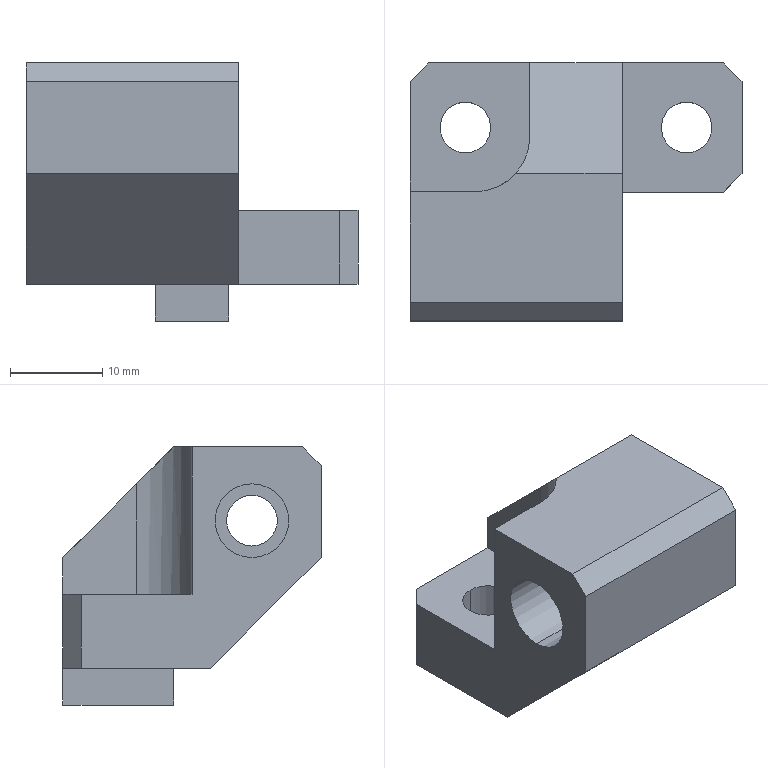Component | SolidWorks | 015GuideRodHolder-1 | 1 solid | 32 faces | box 36 x 28 x 28 mm | volume 10606 mm3 | plane 23 | cylinder 9 | commonest cylinder face diameters 5.5 x6 8 x2 12 x1
build123d program:
from build123d import *

# Parameters (mm, degrees)
SKETCH1_W                = 14
SKETCH1_H                = 36
EXTRUDE1_DEPTH           = 8
SKETCH3_W                = 28
SKETCH3_H                = 10
EXTRUDE3_DEPTH           = 16
M5_CLEARANCE_HOLE2_D     = 5.5
M5_CLEARANCE_HOLE2_DEPTH = 40
SKETCH7_R                = 4
CUT_EXTRUDE1_DEPTH       = 6
M5_CLEARANCE_HOLE1_D     = 5.5
M5_CLEARANCE_HOLE1_DEPTH = 23
SKETCH10_W               = 14
SKETCH10_H               = 10
EXTRUDE4_DEPTH           = 8
BOSS_EXTRUDE1_START      = 13
SKETCH12_W               = 14
SKETCH12_H               = 24
SKETCH12_R               = 4
BOSS_EXTRUDE1_DEPTH      = 13
FILLET1_R                = 6
SKETCH13_W               = 12
SKETCH13_H               = 8
BOSS_EXTRUDE2_DEPTH      = 4
FILLET1_OF_MIRROR3_R     = 6
SKETCH14_W               = 28
SKETCH14_H               = 28
CUT_EXTRUDE2_DEPTH       = 53.545
CHAMFER2_SIZE            = 2
CHAMFER3_SIZE            = 12
CHAMFER4_SIZE            = 2


with BuildPart() as part:
    # Sketch1 → Extrude1 (new body)
    with BuildSketch(Plane.XY):
        Rectangle(SKETCH1_W, SKETCH1_H)
    extrude1 = extrude(amount=EXTRUDE1_DEPTH)

    # Sketch3 → Extrude3 (add)
    with BuildSketch(Plane.XY.offset(8)):
        with Locations((7, 0)):
            Rectangle(SKETCH3_W, SKETCH3_H)
    extrude3 = extrude(amount=EXTRUDE3_DEPTH)

    # M5 Clearance Hole2
    with Locations(Plane.XY.offset(8)):
        with Locations((0, 12), (0, -12)):
            m5_clearance_hole2 = Hole(M5_CLEARANCE_HOLE2_D / 2, depth=M5_CLEARANCE_HOLE2_DEPTH)

    # Sketch7 → Cut-Extrude1 (cut)
    with BuildSketch(Plane(origin=(0, 5, 0), x_dir=(-1, 0, 0), z_dir=(0, 1, 0))):
        with Locations(Location((-13.5, 16, 0), (0, 0, 90))):
            Circle(SKETCH7_R)
    cut_extrude1 = extrude(amount=-CUT_EXTRUDE1_DEPTH, mode=Mode.SUBTRACT)

    # M5 Clearance Hole1
    with Locations(Plane(origin=(13.5, -5, 16), x_dir=(0, 0, -1), z_dir=(0, -1, 0))):
        with Locations((0, 0)):
            m5_clearance_hole1 = Hole(M5_CLEARANCE_HOLE1_D / 2, depth=M5_CLEARANCE_HOLE1_DEPTH)

    # Sketch10 → Extrude4 (add)
    with BuildSketch(Plane(origin=(0, 0, 8), x_dir=(-1, 0, 0), z_dir=(0, 0, -1))):
        with Locations((-14, 0)):
            Rectangle(SKETCH10_W, SKETCH10_H)
    extrude4 = extrude(amount=EXTRUDE4_DEPTH)

    # Sketch12 → Boss-Extrude1 (add)
    with BuildSketch(Plane(origin=(0, 5, 0), x_dir=(1, 0, 0), z_dir=(0, 1, 0)).offset(BOSS_EXTRUDE1_START)):
        with Locations((14, -12)):
            Rectangle(SKETCH12_W, SKETCH12_H)
        with Locations(Location((13.5, -16, 0), (0, 0, 270))):
            Circle(SKETCH12_R, mode=Mode.SUBTRACT)
    boss_extrude1 = extrude(amount=-BOSS_EXTRUDE1_DEPTH)

    # Fillet1
    fillet1_edges = [part.edges().sort_by_distance(p)[0] for p in [
        (7, 5, 16),
    ]]
    fillet(fillet1_edges, radius=FILLET1_R)

    # Sketch13 → Boss-Extrude2 (add)
    with BuildSketch(Plane(origin=(0, 0, 0), x_dir=(-1, 0, 0), z_dir=(0, 0, -1))):
        with Locations((1, 0)):
            Rectangle(SKETCH13_W, SKETCH13_H)
    boss_extrude2 = extrude(amount=BOSS_EXTRUDE2_DEPTH)

    # Mirror3: Extrude1, Extrude3, M5 Clearance Hole2, Cut-Extrude1, M5 Clearance Hole1, Extrude4, Boss-Extrude1, Boss-Extrude2 across plane
    add(extrude1.mirror(Plane.XY.offset(-4)))
    add(extrude3.mirror(Plane.XY.offset(-4)))
    add(m5_clearance_hole2.mirror(Plane.XY.offset(-4)), mode=Mode.SUBTRACT)
    add(cut_extrude1.mirror(Plane.XY.offset(-4)), mode=Mode.SUBTRACT)
    add(m5_clearance_hole1.mirror(Plane.XY.offset(-4)), mode=Mode.SUBTRACT)
    add(extrude4.mirror(Plane.XY.offset(-4)))
    add(boss_extrude1.mirror(Plane.XY.offset(-4)))
    add(boss_extrude2.mirror(Plane.XY.offset(-4)))

    # Fillet1 of Mirror3
    fillet1_of_mirror3_edges = [part.edges().sort_by_distance(p)[0] for p in [
        (7, 5, -24),
    ]]
    fillet(fillet1_of_mirror3_edges, radius=FILLET1_OF_MIRROR3_R)

    # Sketch14 → Cut-Extrude2 (cut, through all)
    with BuildSketch(Plane.XZ.offset(18)):
        with Locations((7, 10)):
            Rectangle(SKETCH14_W, SKETCH14_H)
    extrude(amount=-CUT_EXTRUDE2_DEPTH, mode=Mode.SUBTRACT)

    # Chamfer2
    chamfer2_edges = [part.edges().sort_by_distance(p)[0] for p in [
        (-7, 18, -12),
        (7, -18, -12),
        (-7, -18, -12),
    ]]
    chamfer(chamfer2_edges, length=CHAMFER2_SIZE)

    # Chamfer3
    chamfer3_edges = [part.edges().sort_by_distance(p)[0] for p in [
        (21, 6.5, -8),
        (-7, 0, -32),
    ]]
    chamfer(chamfer3_edges, length=CHAMFER3_SIZE)

    # Chamfer4
    chamfer4_edges = [part.edges().sort_by_distance(p)[0] for p in [
        (21, 6.5, -32),
    ]]
    chamfer(chamfer4_edges, length=CHAMFER4_SIZE)


solid = part.part

# Placed as in the assembly
solid = solid.moved(Location((25.76, 38.424, 29.04), (180, 0, 90)))
STEP:
#1=COLOUR_RGB('',0.7922,0.8196,0.9333);
#2=FILL_AREA_STYLE_COLOUR('',#1);
#3=FILL_AREA_STYLE('',(#2));
#4=SURFACE_STYLE_FILL_AREA(#3);
#5=SURFACE_SIDE_STYLE('',(#4));
#6=SURFACE_STYLE_USAGE(.BOTH.,#5);
#7=PRESENTATION_STYLE_ASSIGNMENT((#6));
#8=CARTESIAN_POINT('',(1.054,0.9813,2.196));
#9=VERTEX_POINT('',#8);
#10=CARTESIAN_POINT('',(1.054,0.9813,1.98));
#11=VERTEX_POINT('',#10);
#12=CARTESIAN_POINT('',(1.054,0.9813,2.088));
#13=DIRECTION('',(1.,0.,0.));
#14=DIRECTION('',(0.,0.,1.));
#15=AXIS2_PLACEMENT_3D('',#12,#13,#14);
#16=CIRCLE('',#15,0.1083);
#17=EDGE_CURVE('',#9,#11,#16,.T.);
#18=ORIENTED_EDGE('',*,*,#17,.F.);
#19=CARTESIAN_POINT('',(1.211,0.9813,2.196));
#20=VERTEX_POINT('',#19);
#21=CARTESIAN_POINT('',(1.211,0.9813,2.196));
#22=DIRECTION('',(1.,0.,0.));
#23=VECTOR('',#22,39.37);
#24=LINE('',#21,#23);
#25=EDGE_CURVE('',#9,#20,#24,.T.);
#26=ORIENTED_EDGE('',*,*,#25,.T.);
#27=CARTESIAN_POINT('',(1.211,0.9813,1.98));
#28=VERTEX_POINT('',#27);
#29=CARTESIAN_POINT('',(1.211,0.9813,2.088));
#30=DIRECTION('',(-1.,-0.,0.));
#31=DIRECTION('',(0.,0.,-1.));
#32=AXIS2_PLACEMENT_3D('',#29,#30,#31);
#33=CIRCLE('',#32,0.1083);
#34=EDGE_CURVE('',#28,#20,#33,.T.);
#35=ORIENTED_EDGE('',*,*,#34,.F.);
#36=CARTESIAN_POINT('',(1.211,0.9813,1.98));
#37=DIRECTION('',(1.,0.,0.));
#38=VECTOR('',#37,39.37);
#39=LINE('',#36,#38);
#40=EDGE_CURVE('',#11,#28,#39,.T.);
#41=ORIENTED_EDGE('',*,*,#40,.F.);
#42=EDGE_LOOP('',(#18,#26,#35,#41));
#43=FACE_OUTER_BOUND('',#42,.T.);
#44=CARTESIAN_POINT('',(1.211,0.9813,2.088));
#45=DIRECTION('',(1.,0.,0.));
#46=DIRECTION('',(0.,0.,-1.));
#47=AXIS2_PLACEMENT_3D('',#44,#45,#46);
#48=CYLINDRICAL_SURFACE('',#47,0.1083);
#49=ADVANCED_FACE('',(#43),#48,.F.);
#50=CARTESIAN_POINT('',(1.054,0.9813,2.246));
#51=VERTEX_POINT('',#50);
#52=CARTESIAN_POINT('',(1.054,0.9813,1.931));
#53=VERTEX_POINT('',#52);
#54=CARTESIAN_POINT('',(1.054,0.9813,2.088));
#55=DIRECTION('',(1.,0.,0.));
#56=DIRECTION('',(0.,0.,1.));
#57=AXIS2_PLACEMENT_3D('',#54,#55,#56);
#58=CIRCLE('',#57,0.1575);
#59=EDGE_CURVE('',#51,#53,#58,.T.);
#60=ORIENTED_EDGE('',*,*,#59,.T.);
#61=CARTESIAN_POINT('',(0.3055,0.9813,1.931));
#62=VERTEX_POINT('',#61);
#63=CARTESIAN_POINT('',(1.054,0.9813,1.931));
#64=DIRECTION('',(-1.,-0.,0.));
#65=VECTOR('',#64,39.37);
#66=LINE('',#63,#65);
#67=EDGE_CURVE('',#53,#62,#66,.T.);
#68=ORIENTED_EDGE('',*,*,#67,.T.);
#69=CARTESIAN_POINT('',(0.3055,0.9813,2.246));
#70=VERTEX_POINT('',#69);
#71=CARTESIAN_POINT('',(0.3055,0.9813,2.088));
#72=DIRECTION('',(-1.,-0.,0.));
#73=DIRECTION('',(-0.,0.,-1.));
#74=AXIS2_PLACEMENT_3D('',#71,#72,#73);
#75=CIRCLE('',#74,0.1575);
#76=EDGE_CURVE('',#62,#70,#75,.T.);
#77=ORIENTED_EDGE('',*,*,#76,.T.);
#78=CARTESIAN_POINT('',(1.054,0.9813,2.246));
#79=DIRECTION('',(-1.,-0.,0.));
#80=VECTOR('',#79,39.37);
#81=LINE('',#78,#80);
#82=EDGE_CURVE('',#51,#70,#81,.T.);
#83=ORIENTED_EDGE('',*,*,#82,.F.);
#84=EDGE_LOOP('',(#60,#68,#77,#83));
#85=FACE_OUTER_BOUND('',#84,.T.);
#86=CARTESIAN_POINT('',(1.054,0.9813,2.088));
#87=DIRECTION('',(-1.,-0.,0.));
#88=DIRECTION('',(0.,0.,1.));
#89=AXIS2_PLACEMENT_3D('',#86,#87,#88);
#90=CYLINDRICAL_SURFACE('',#89,0.1575);
#91=ADVANCED_FACE('',(#85),#90,.F.);
#92=CARTESIAN_POINT('',(0.5417,1.405,1.458));
#93=VERTEX_POINT('',#92);
#94=CARTESIAN_POINT('',(0.5417,1.621,1.458));
#95=VERTEX_POINT('',#94);
#96=CARTESIAN_POINT('',(0.5417,1.513,1.458));
#97=DIRECTION('',(-0.,0.,-1.));
#98=DIRECTION('',(0.,-1.,0.));
#99=AXIS2_PLACEMENT_3D('',#96,#97,#98);
#100=CIRCLE('',#99,0.1083);
#101=EDGE_CURVE('',#93,#95,#100,.T.);
#102=ORIENTED_EDGE('',*,*,#101,.T.);
#103=CARTESIAN_POINT('',(0.5417,1.621,1.773));
#104=VERTEX_POINT('',#103);
#105=CARTESIAN_POINT('',(0.5417,1.621,1.773));
#106=DIRECTION('',(0.,-0.,1.));
#107=VECTOR('',#106,39.37);
#108=LINE('',#105,#107);
#109=EDGE_CURVE('',#95,#104,#108,.T.);
#110=ORIENTED_EDGE('',*,*,#109,.T.);
#111=CARTESIAN_POINT('',(0.5417,1.405,1.773));
#112=VERTEX_POINT('',#111);
#113=CARTESIAN_POINT('',(0.5417,1.513,1.773));
#114=DIRECTION('',(-0.,0.,-1.));
#115=DIRECTION('',(0.,-1.,0.));
#116=AXIS2_PLACEMENT_3D('',#113,#114,#115);
#117=CIRCLE('',#116,0.1083);
#118=EDGE_CURVE('',#112,#104,#117,.T.);
#119=ORIENTED_EDGE('',*,*,#118,.F.);
#120=CARTESIAN_POINT('',(0.5417,1.405,1.773));
#121=DIRECTION('',(0.,-0.,1.));
#122=VECTOR('',#121,39.37);
#123=LINE('',#120,#122);
#124=EDGE_CURVE('',#93,#112,#123,.T.);
#125=ORIENTED_EDGE('',*,*,#124,.F.);
#126=EDGE_LOOP('',(#102,#110,#119,#125));
#127=FACE_OUTER_BOUND('',#126,.T.);
#128=CARTESIAN_POINT('',(0.5417,1.513,1.773));
#129=DIRECTION('',(0.,-0.,1.));
#130=DIRECTION('',(0.,-1.,0.));
#131=AXIS2_PLACEMENT_3D('',#128,#129,#130);
#132=CYLINDRICAL_SURFACE('',#131,0.1083);
#133=ADVANCED_FACE('',(#127),#132,.F.);
#134=CARTESIAN_POINT('',(1.487,1.405,1.458));
#135=VERTEX_POINT('',#134);
#136=CARTESIAN_POINT('',(1.487,1.621,1.458));
#137=VERTEX_POINT('',#136);
#138=CARTESIAN_POINT('',(1.487,1.513,1.458));
#139=DIRECTION('',(-0.,0.,-1.));
#140=DIRECTION('',(0.,-1.,0.));
#141=AXIS2_PLACEMENT_3D('',#138,#139,#140);
#142=CIRCLE('',#141,0.1083);
#143=EDGE_CURVE('',#135,#137,#142,.T.);
#144=ORIENTED_EDGE('',*,*,#143,.T.);
#145=CARTESIAN_POINT('',(1.487,1.621,1.773));
#146=VERTEX_POINT('',#145);
#147=CARTESIAN_POINT('',(1.487,1.621,1.773));
#148=DIRECTION('',(0.,-0.,1.));
#149=VECTOR('',#148,39.37);
#150=LINE('',#147,#149);
#151=EDGE_CURVE('',#137,#146,#150,.T.);
#152=ORIENTED_EDGE('',*,*,#151,.T.);
#153=CARTESIAN_POINT('',(1.487,1.405,1.773));
#154=VERTEX_POINT('',#153);
#155=CARTESIAN_POINT('',(1.487,1.513,1.773));
#156=DIRECTION('',(-0.,0.,-1.));
#157=DIRECTION('',(0.,-1.,0.));
#158=AXIS2_PLACEMENT_3D('',#155,#156,#157);
#159=CIRCLE('',#158,0.1083);
#160=EDGE_CURVE('',#154,#146,#159,.T.);
#161=ORIENTED_EDGE('',*,*,#160,.F.);
#162=CARTESIAN_POINT('',(1.487,1.405,1.773));
#163=DIRECTION('',(0.,-0.,1.));
#164=VECTOR('',#163,39.37);
#165=LINE('',#162,#164);
#166=EDGE_CURVE('',#135,#154,#165,.T.);
#167=ORIENTED_EDGE('',*,*,#166,.F.);
#168=EDGE_LOOP('',(#144,#152,#161,#167));
#169=FACE_OUTER_BOUND('',#168,.T.);
#170=CARTESIAN_POINT('',(1.487,1.513,1.773));
#171=DIRECTION('',(0.,-0.,1.));
#172=DIRECTION('',(0.,-1.,0.));
#173=AXIS2_PLACEMENT_3D('',#170,#171,#172);
#174=CYLINDRICAL_SURFACE('',#173,0.1083);
#175=ADVANCED_FACE('',(#169),#174,.F.);
#176=CARTESIAN_POINT('',(0.8173,1.788,1.931));
#177=VERTEX_POINT('',#176);
#178=CARTESIAN_POINT('',(0.8173,1.788,1.773));
#179=VERTEX_POINT('',#178);
#180=CARTESIAN_POINT('',(0.8173,1.788,2.403));
#181=DIRECTION('',(-0.,0.,-1.));
#182=VECTOR('',#181,39.37);
#183=LINE('',#180,#182);
#184=EDGE_CURVE('',#177,#179,#183,.T.);
#185=ORIENTED_EDGE('',*,*,#184,.F.);
#186=CARTESIAN_POINT('',(1.211,1.788,1.931));
#187=VERTEX_POINT('',#186);
#188=CARTESIAN_POINT('',(1.211,1.788,1.931));
#189=DIRECTION('',(1.,-0.,-0.));
#190=VECTOR('',#189,39.37);
#191=LINE('',#188,#190);
#192=EDGE_CURVE('',#177,#187,#191,.T.);
#193=ORIENTED_EDGE('',*,*,#192,.T.);
#194=CARTESIAN_POINT('',(1.211,1.788,1.773));
#195=VERTEX_POINT('',#194);
#196=CARTESIAN_POINT('',(1.211,1.788,2.403));
#197=DIRECTION('',(-0.,0.,-1.));
#198=VECTOR('',#197,39.37);
#199=LINE('',#196,#198);
#200=EDGE_CURVE('',#187,#195,#199,.T.);
#201=ORIENTED_EDGE('',*,*,#200,.T.);
#202=CARTESIAN_POINT('',(1.644,1.788,1.773));
#203=VERTEX_POINT('',#202);
#204=CARTESIAN_POINT('',(0.3055,1.788,1.773));
#205=DIRECTION('',(1.,-0.,-0.));
#206=VECTOR('',#205,39.37);
#207=LINE('',#204,#206);
#208=EDGE_CURVE('',#195,#203,#207,.T.);
#209=ORIENTED_EDGE('',*,*,#208,.T.);
#210=CARTESIAN_POINT('',(1.644,1.788,1.458));
#211=VERTEX_POINT('',#210);
#212=CARTESIAN_POINT('',(1.644,1.788,0.8284));
#213=DIRECTION('',(-0.,0.,-1.));
#214=VECTOR('',#213,39.37);
#215=LINE('',#212,#214);
#216=EDGE_CURVE('',#203,#211,#215,.T.);
#217=ORIENTED_EDGE('',*,*,#216,.T.);
#218=CARTESIAN_POINT('',(1.172,1.788,1.458));
#219=VERTEX_POINT('',#218);
#220=CARTESIAN_POINT('',(0.3055,1.788,1.458));
#221=DIRECTION('',(1.,-0.,-0.));
#222=VECTOR('',#221,39.37);
#223=LINE('',#220,#222);
#224=EDGE_CURVE('',#219,#211,#223,.T.);
#225=ORIENTED_EDGE('',*,*,#224,.F.);
#226=CARTESIAN_POINT('',(1.172,1.788,1.301));
#227=VERTEX_POINT('',#226);
#228=CARTESIAN_POINT('',(1.172,1.788,1.301));
#229=DIRECTION('',(-0.,0.,-1.));
#230=VECTOR('',#229,39.37);
#231=LINE('',#228,#230);
#232=EDGE_CURVE('',#219,#227,#231,.T.);
#233=ORIENTED_EDGE('',*,*,#232,.T.);
#234=CARTESIAN_POINT('',(0.8567,1.788,1.301));
#235=VERTEX_POINT('',#234);
#236=CARTESIAN_POINT('',(0.3055,1.788,1.301));
#237=DIRECTION('',(1.,0.,0.));
#238=VECTOR('',#237,39.37);
#239=LINE('',#236,#238);
#240=EDGE_CURVE('',#235,#227,#239,.T.);
#241=ORIENTED_EDGE('',*,*,#240,.F.);
#242=CARTESIAN_POINT('',(0.8567,1.788,1.458));
#243=VERTEX_POINT('',#242);
#244=CARTESIAN_POINT('',(0.8567,1.788,1.301));
#245=DIRECTION('',(-0.,0.,-1.));
#246=VECTOR('',#245,39.37);
#247=LINE('',#244,#246);
#248=EDGE_CURVE('',#243,#235,#247,.T.);
#249=ORIENTED_EDGE('',*,*,#248,.F.);
#250=CARTESIAN_POINT('',(0.3842,1.788,1.458));
#251=VERTEX_POINT('',#250);
#252=CARTESIAN_POINT('',(0.3055,1.788,1.458));
#253=DIRECTION('',(1.,-0.,-0.));
#254=VECTOR('',#253,39.37);
#255=LINE('',#252,#254);
#256=EDGE_CURVE('',#251,#243,#255,.T.);
#257=ORIENTED_EDGE('',*,*,#256,.F.);
#258=CARTESIAN_POINT('',(0.3842,1.788,1.773));
#259=VERTEX_POINT('',#258);
#260=CARTESIAN_POINT('',(0.3842,1.788,0.8284));
#261=DIRECTION('',(0.,-0.,1.));
#262=VECTOR('',#261,39.37);
#263=LINE('',#260,#262);
#264=EDGE_CURVE('',#251,#259,#263,.T.);
#265=ORIENTED_EDGE('',*,*,#264,.T.);
#266=CARTESIAN_POINT('',(0.3055,1.788,1.773));
#267=DIRECTION('',(1.,-0.,-0.));
#268=VECTOR('',#267,39.37);
#269=LINE('',#266,#268);
#270=EDGE_CURVE('',#259,#179,#269,.T.);
#271=ORIENTED_EDGE('',*,*,#270,.T.);
#272=EDGE_LOOP('',(#185,#193,#201,#209,#217,#225,#233,#241,#249,#257,#265,#271));
#273=FACE_OUTER_BOUND('',#272,.T.);
#274=CARTESIAN_POINT('',(0.3055,1.788,0.8284));
#275=DIRECTION('',(-0.,-1.,-0.));
#276=DIRECTION('',(-1.,0.,0.));
#277=AXIS2_PLACEMENT_3D('',#274,#275,#276);
#278=PLANE('',#277);
#279=ADVANCED_FACE('',(#273),#278,.F.);
#280=ORIENTED_EDGE('',*,*,#248,.T.);
#281=CARTESIAN_POINT('',(0.8567,1.316,1.301));
#282=VERTEX_POINT('',#281);
#283=CARTESIAN_POINT('',(0.8567,1.788,1.301));
#284=DIRECTION('',(0.,-1.,-0.));
#285=VECTOR('',#284,39.37);
#286=LINE('',#283,#285);
#287=EDGE_CURVE('',#235,#282,#286,.T.);
#288=ORIENTED_EDGE('',*,*,#287,.T.);
#289=CARTESIAN_POINT('',(0.8567,1.316,1.458));
#290=VERTEX_POINT('',#289);
#291=CARTESIAN_POINT('',(0.8567,1.316,1.301));
#292=DIRECTION('',(-0.,0.,-1.));
#293=VECTOR('',#292,39.37);
#294=LINE('',#291,#293);
#295=EDGE_CURVE('',#290,#282,#294,.T.);
#296=ORIENTED_EDGE('',*,*,#295,.F.);
#297=CARTESIAN_POINT('',(0.8567,1.788,1.458));
#298=DIRECTION('',(0.,-1.,-0.));
#299=VECTOR('',#298,39.37);
#300=LINE('',#297,#299);
#301=EDGE_CURVE('',#243,#290,#300,.T.);
#302=ORIENTED_EDGE('',*,*,#301,.F.);
#303=EDGE_LOOP('',(#280,#288,#296,#302));
#304=FACE_OUTER_BOUND('',#303,.T.);
#305=CARTESIAN_POINT('',(0.8567,1.788,1.301));
#306=DIRECTION('',(1.,0.,0.));
#307=DIRECTION('',(0.,-1.,-0.));
#308=AXIS2_PLACEMENT_3D('',#305,#306,#307);
#309=PLANE('',#308);
#310=ADVANCED_FACE('',(#304),#309,.F.);
#311=ORIENTED_EDGE('',*,*,#295,.T.);
#312=CARTESIAN_POINT('',(1.172,1.316,1.301));
#313=VERTEX_POINT('',#312);
#314=CARTESIAN_POINT('',(0.8567,1.316,1.301));
#315=DIRECTION('',(1.,0.,0.));
#316=VECTOR('',#315,39.37);
#317=LINE('',#314,#316);
#318=EDGE_CURVE('',#282,#313,#317,.T.);
#319=ORIENTED_EDGE('',*,*,#318,.T.);
#320=CARTESIAN_POINT('',(1.172,1.316,1.458));
#321=VERTEX_POINT('',#320);
#322=CARTESIAN_POINT('',(1.172,1.316,1.301));
#323=DIRECTION('',(-0.,0.,-1.));
#324=VECTOR('',#323,39.37);
#325=LINE('',#322,#324);
#326=EDGE_CURVE('',#321,#313,#325,.T.);
#327=ORIENTED_EDGE('',*,*,#326,.F.);
#328=CARTESIAN_POINT('',(0.8567,1.316,1.458));
#329=DIRECTION('',(1.,0.,0.));
#330=VECTOR('',#329,39.37);
#331=LINE('',#328,#330);
#332=EDGE_CURVE('',#290,#321,#331,.T.);
#333=ORIENTED_EDGE('',*,*,#332,.F.);
#334=EDGE_LOOP('',(#311,#319,#327,#333));
#335=FACE_OUTER_BOUND('',#334,.T.);
#336=CARTESIAN_POINT('',(0.8567,1.316,1.301));
#337=DIRECTION('',(-0.,1.,0.));
#338=DIRECTION('',(1.,0.,0.));
#339=AXIS2_PLACEMENT_3D('',#336,#337,#338);
#340=PLANE('',#339);
#341=ADVANCED_FACE('',(#335),#340,.F.);
#342=ORIENTED_EDGE('',*,*,#326,.T.);
#343=CARTESIAN_POINT('',(1.172,1.788,1.301));
#344=DIRECTION('',(-0.,1.,0.));
#345=VECTOR('',#344,39.37);
#346=LINE('',#343,#345);
#347=EDGE_CURVE('',#313,#227,#346,.T.);
#348=ORIENTED_EDGE('',*,*,#347,.T.);
#349=ORIENTED_EDGE('',*,*,#232,.F.);
#350=CARTESIAN_POINT('',(1.172,1.788,1.458));
#351=DIRECTION('',(-0.,1.,0.));
#352=VECTOR('',#351,39.37);
#353=LINE('',#350,#352);
#354=EDGE_CURVE('',#321,#219,#353,.T.);
#355=ORIENTED_EDGE('',*,*,#354,.F.);
#356=EDGE_LOOP('',(#342,#348,#349,#355));
#357=FACE_OUTER_BOUND('',#356,.T.);
#358=CARTESIAN_POINT('',(1.172,1.788,1.301));
#359=DIRECTION('',(-1.,-0.,-0.));
#360=DIRECTION('',(-0.,1.,0.));
#361=AXIS2_PLACEMENT_3D('',#358,#359,#360);
#362=PLANE('',#361);
#363=ADVANCED_FACE('',(#357),#362,.F.);
#364=ORIENTED_EDGE('',*,*,#143,.F.);
#365=CARTESIAN_POINT('',(1.487,1.513,1.458));
#366=DIRECTION('',(-0.,0.,-1.));
#367=DIRECTION('',(0.,-1.,0.));
#368=AXIS2_PLACEMENT_3D('',#365,#366,#367);
#369=CIRCLE('',#368,0.1083);
#370=EDGE_CURVE('',#137,#135,#369,.T.);
#371=ORIENTED_EDGE('',*,*,#370,.F.);
#372=EDGE_LOOP('',(#364,#371));
#373=FACE_BOUND('',#372,.T.);
#374=ORIENTED_EDGE('',*,*,#101,.F.);
#375=CARTESIAN_POINT('',(0.5417,1.513,1.458));
#376=DIRECTION('',(-0.,0.,-1.));
#377=DIRECTION('',(0.,-1.,0.));
#378=AXIS2_PLACEMENT_3D('',#375,#376,#377);
#379=CIRCLE('',#378,0.1083);
#380=EDGE_CURVE('',#95,#93,#379,.T.);
#381=ORIENTED_EDGE('',*,*,#380,.F.);
#382=EDGE_LOOP('',(#374,#381));
#383=FACE_BOUND('',#382,.T.);
#384=CARTESIAN_POINT('',(1.211,1.158,1.458));
#385=VERTEX_POINT('',#384);
#386=CARTESIAN_POINT('',(1.211,1.237,1.458));
#387=VERTEX_POINT('',#386);
#388=CARTESIAN_POINT('',(1.211,0.686,1.458));
#389=DIRECTION('',(-0.,1.,0.));
#390=VECTOR('',#389,39.37);
#391=LINE('',#388,#390);
#392=EDGE_CURVE('',#385,#387,#391,.T.);
#393=ORIENTED_EDGE('',*,*,#392,.F.);
#394=CARTESIAN_POINT('',(0.3055,1.158,1.458));
#395=VERTEX_POINT('',#394);
#396=CARTESIAN_POINT('',(1.723,1.158,1.458));
#397=DIRECTION('',(-1.,-0.,0.));
#398=VECTOR('',#397,39.37);
#399=LINE('',#396,#398);
#400=EDGE_CURVE('',#385,#395,#399,.T.);
#401=ORIENTED_EDGE('',*,*,#400,.T.);
#402=CARTESIAN_POINT('',(0.3055,1.71,1.458));
#403=VERTEX_POINT('',#402);
#404=CARTESIAN_POINT('',(0.3055,1.788,1.458));
#405=DIRECTION('',(-0.,1.,0.));
#406=VECTOR('',#405,39.37);
#407=LINE('',#404,#406);
#408=EDGE_CURVE('',#395,#403,#407,.T.);
#409=ORIENTED_EDGE('',*,*,#408,.T.);
#410=CARTESIAN_POINT('',(0.3055,1.71,1.458));
#411=DIRECTION('',(0.7071,0.7071,0.));
#412=VECTOR('',#411,39.37);
#413=LINE('',#410,#412);
#414=EDGE_CURVE('',#403,#251,#413,.T.);
#415=ORIENTED_EDGE('',*,*,#414,.T.);
#416=ORIENTED_EDGE('',*,*,#256,.T.);
#417=ORIENTED_EDGE('',*,*,#301,.T.);
#418=ORIENTED_EDGE('',*,*,#332,.T.);
#419=ORIENTED_EDGE('',*,*,#354,.T.);
#420=ORIENTED_EDGE('',*,*,#224,.T.);
#421=CARTESIAN_POINT('',(1.723,1.71,1.458));
#422=VERTEX_POINT('',#421);
#423=CARTESIAN_POINT('',(1.644,1.788,1.458));
#424=DIRECTION('',(0.7071,-0.7071,-0.));
#425=VECTOR('',#424,39.37);
#426=LINE('',#423,#425);
#427=EDGE_CURVE('',#211,#422,#426,.T.);
#428=ORIENTED_EDGE('',*,*,#427,.T.);
#429=CARTESIAN_POINT('',(1.723,1.316,1.458));
#430=VERTEX_POINT('',#429);
#431=CARTESIAN_POINT('',(1.723,1.788,1.458));
#432=DIRECTION('',(0.,-1.,-0.));
#433=VECTOR('',#432,39.37);
#434=LINE('',#431,#433);
#435=EDGE_CURVE('',#422,#430,#434,.T.);
#436=ORIENTED_EDGE('',*,*,#435,.T.);
#437=CARTESIAN_POINT('',(1.644,1.237,1.458));
#438=VERTEX_POINT('',#437);
#439=CARTESIAN_POINT('',(1.723,1.316,1.458));
#440=DIRECTION('',(-0.7071,-0.7071,-0.));
#441=VECTOR('',#440,39.37);
#442=LINE('',#439,#441);
#443=EDGE_CURVE('',#430,#438,#442,.T.);
#444=ORIENTED_EDGE('',*,*,#443,.T.);
#445=CARTESIAN_POINT('',(0.3055,1.237,1.458));
#446=DIRECTION('',(-1.,0.,0.));
#447=VECTOR('',#446,39.37);
#448=LINE('',#445,#447);
#449=EDGE_CURVE('',#438,#387,#448,.T.);
#450=ORIENTED_EDGE('',*,*,#449,.T.);
#451=EDGE_LOOP('',(#393,#401,#409,#415,#416,#417,#418,#419,#420,#428,#436,#444,#450));
#452=FACE_OUTER_BOUND('',#451,.T.);
#453=CARTESIAN_POINT('',(1.723,1.788,1.458));
#454=DIRECTION('',(0.,-0.,1.));
#455=DIRECTION('',(0.,-1.,-0.));
#456=AXIS2_PLACEMENT_3D('',#453,#454,#455);
#457=PLANE('',#456);
#458=ADVANCED_FACE('',(#373,#383,#452),#457,.F.);
#459=CARTESIAN_POINT('',(0.8173,1.473,2.246));
#460=VERTEX_POINT('',#459);
#461=CARTESIAN_POINT('',(0.8173,1.473,1.773));
#462=VERTEX_POINT('',#461);
#463=CARTESIAN_POINT('',(0.8173,1.473,1.773));
#464=DIRECTION('',(-0.,0.,-1.));
#465=VECTOR('',#464,39.37);
#466=LINE('',#463,#465);
#467=EDGE_CURVE('',#460,#462,#466,.T.);
#468=ORIENTED_EDGE('',*,*,#467,.F.);
#469=CARTESIAN_POINT('',(0.8173,1.788,1.931));
#470=DIRECTION('',(-0.,0.7071,-0.7071));
#471=VECTOR('',#470,39.37);
#472=LINE('',#469,#471);
#473=EDGE_CURVE('',#460,#177,#472,.T.);
#474=ORIENTED_EDGE('',*,*,#473,.T.);
#475=ORIENTED_EDGE('',*,*,#184,.T.);
#476=CARTESIAN_POINT('',(0.8173,1.788,1.773));
#477=DIRECTION('',(-0.,1.,0.));
#478=VECTOR('',#477,39.37);
#479=LINE('',#476,#478);
#480=EDGE_CURVE('',#462,#179,#479,.T.);
#481=ORIENTED_EDGE('',*,*,#480,.F.);
#482=EDGE_LOOP('',(#468,#474,#475,#481));
#483=FACE_OUTER_BOUND('',#482,.T.);
#484=CARTESIAN_POINT('',(0.8173,1.788,2.403));
#485=DIRECTION('',(1.,0.,-0.));
#486=DIRECTION('',(-0.,0.,-1.));
#487=AXIS2_PLACEMENT_3D('',#484,#485,#486);
#488=PLANE('',#487);
#489=ADVANCED_FACE('',(#483),#488,.F.);
#490=ORIENTED_EDGE('',*,*,#449,.F.);
#491=CARTESIAN_POINT('',(1.644,1.237,1.773));
#492=VERTEX_POINT('',#491);
#493=CARTESIAN_POINT('',(1.644,1.237,1.773));
#494=DIRECTION('',(0.,-0.,1.));
#495=VECTOR('',#494,39.37);
#496=LINE('',#493,#495);
#497=EDGE_CURVE('',#438,#492,#496,.T.);
#498=ORIENTED_EDGE('',*,*,#497,.T.);
#499=CARTESIAN_POINT('',(1.211,1.237,1.773));
#500=VERTEX_POINT('',#499);
#501=CARTESIAN_POINT('',(0.3055,1.237,1.773));
#502=DIRECTION('',(-1.,0.,0.));
#503=VECTOR('',#502,39.37);
#504=LINE('',#501,#503);
#505=EDGE_CURVE('',#492,#500,#504,.T.);
#506=ORIENTED_EDGE('',*,*,#505,.T.);
#507=CARTESIAN_POINT('',(1.211,1.237,1.458));
#508=DIRECTION('',(0.,-0.,1.));
#509=VECTOR('',#508,39.37);
#510=LINE('',#507,#509);
#511=EDGE_CURVE('',#387,#500,#510,.T.);
#512=ORIENTED_EDGE('',*,*,#511,.F.);
#513=EDGE_LOOP('',(#490,#498,#506,#512));
#514=FACE_OUTER_BOUND('',#513,.T.);
#515=CARTESIAN_POINT('',(0.3055,1.237,1.773));
#516=DIRECTION('',(0.,1.,0.));
#517=DIRECTION('',(1.,-0.,-0.));
#518=AXIS2_PLACEMENT_3D('',#515,#516,#517);
#519=PLANE('',#518);
#520=ADVANCED_FACE('',(#514),#519,.F.);
#521=ORIENTED_EDGE('',*,*,#118,.T.);
#522=CARTESIAN_POINT('',(0.5417,1.513,1.773));
#523=DIRECTION('',(-0.,0.,-1.));
#524=DIRECTION('',(0.,-1.,0.));
#525=AXIS2_PLACEMENT_3D('',#522,#523,#524);
#526=CIRCLE('',#525,0.1083);
#527=EDGE_CURVE('',#104,#112,#526,.T.);
#528=ORIENTED_EDGE('',*,*,#527,.T.);
#529=EDGE_LOOP('',(#521,#528));
#530=FACE_BOUND('',#529,.T.);
#531=ORIENTED_EDGE('',*,*,#270,.F.);
#532=CARTESIAN_POINT('',(0.3055,1.71,1.773));
#533=VERTEX_POINT('',#532);
#534=CARTESIAN_POINT('',(1.054,2.458,1.773));
#535=DIRECTION('',(-0.7071,-0.7071,-0.));
#536=VECTOR('',#535,39.37);
#537=LINE('',#534,#536);
#538=EDGE_CURVE('',#259,#533,#537,.T.);
#539=ORIENTED_EDGE('',*,*,#538,.T.);
#540=CARTESIAN_POINT('',(0.3055,1.237,1.773));
#541=VERTEX_POINT('',#540);
#542=CARTESIAN_POINT('',(0.3055,1.788,1.773));
#543=DIRECTION('',(-0.,1.,0.));
#544=VECTOR('',#543,39.37);
#545=LINE('',#542,#544);
#546=EDGE_CURVE('',#541,#533,#545,.T.);
#547=ORIENTED_EDGE('',*,*,#546,.F.);
#548=CARTESIAN_POINT('',(0.5811,1.237,1.773));
#549=VERTEX_POINT('',#548);
#550=CARTESIAN_POINT('',(0.3055,1.237,1.773));
#551=DIRECTION('',(-1.,0.,0.));
#552=VECTOR('',#551,39.37);
#553=LINE('',#550,#552);
#554=EDGE_CURVE('',#549,#541,#553,.T.);
#555=ORIENTED_EDGE('',*,*,#554,.F.);
#556=CARTESIAN_POINT('',(0.5811,1.473,1.773));
#557=DIRECTION('',(-0.,0.,-1.));
#558=DIRECTION('',(0.,-1.,0.));
#559=AXIS2_PLACEMENT_3D('',#556,#557,#558);
#560=CIRCLE('',#559,0.2362);
#561=EDGE_CURVE('',#462,#549,#560,.T.);
#562=ORIENTED_EDGE('',*,*,#561,.F.);
#563=ORIENTED_EDGE('',*,*,#480,.T.);
#564=EDGE_LOOP('',(#531,#539,#547,#555,#562,#563));
#565=FACE_OUTER_BOUND('',#564,.T.);
#566=CARTESIAN_POINT('',(1.723,1.788,1.773));
#567=DIRECTION('',(0.,-0.,1.));
#568=DIRECTION('',(0.,-1.,-0.));
#569=AXIS2_PLACEMENT_3D('',#566,#567,#568);
#570=PLANE('',#569);
#571=ADVANCED_FACE('',(#530,#565),#570,.T.);
#572=CARTESIAN_POINT('',(1.723,1.71,1.773));
#573=VERTEX_POINT('',#572);
#574=CARTESIAN_POINT('',(1.723,1.316,1.773));
#575=VERTEX_POINT('',#574);
#576=CARTESIAN_POINT('',(1.723,1.788,1.773));
#577=DIRECTION('',(0.,-1.,-0.));
#578=VECTOR('',#577,39.37);
#579=LINE('',#576,#578);
#580=EDGE_CURVE('',#573,#575,#579,.T.);
#581=ORIENTED_EDGE('',*,*,#580,.T.);
#582=CARTESIAN_POINT('',(1.723,1.316,1.773));
#583=DIRECTION('',(-0.,0.,-1.));
#584=VECTOR('',#583,39.37);
#585=LINE('',#582,#584);
#586=EDGE_CURVE('',#575,#430,#585,.T.);
#587=ORIENTED_EDGE('',*,*,#586,.T.);
#588=ORIENTED_EDGE('',*,*,#435,.F.);
#589=CARTESIAN_POINT('',(1.723,1.71,1.773));
#590=DIRECTION('',(0.,-0.,1.));
#591=VECTOR('',#590,39.37);
#592=LINE('',#589,#591);
#593=EDGE_CURVE('',#422,#573,#592,.T.);
#594=ORIENTED_EDGE('',*,*,#593,.T.);
#595=EDGE_LOOP('',(#581,#587,#588,#594));
#596=FACE_OUTER_BOUND('',#595,.T.);
#597=CARTESIAN_POINT('',(1.723,1.788,1.773));
#598=DIRECTION('',(-1.,-0.,0.));
#599=DIRECTION('',(0.,-0.,1.));
#600=AXIS2_PLACEMENT_3D('',#597,#598,#599);
#601=PLANE('',#600);
#602=ADVANCED_FACE('',(#596),#601,.F.);
#603=CARTESIAN_POINT('',(0.3055,0.686,1.931));
#604=VERTEX_POINT('',#603);
#605=CARTESIAN_POINT('',(0.3055,0.686,2.324));
#606=VERTEX_POINT('',#605);
#607=CARTESIAN_POINT('',(0.3055,0.686,1.458));
#608=DIRECTION('',(0.,-0.,1.));
#609=VECTOR('',#608,39.37);
#610=LINE('',#607,#609);
#611=EDGE_CURVE('',#604,#606,#610,.T.);
#612=ORIENTED_EDGE('',*,*,#611,.T.);
#613=CARTESIAN_POINT('',(0.3055,0.7647,2.403));
#614=VERTEX_POINT('',#613);
#615=CARTESIAN_POINT('',(0.3055,0.686,2.324));
#616=DIRECTION('',(0.,0.7071,0.7071));
#617=VECTOR('',#616,39.37);
#618=LINE('',#615,#617);
#619=EDGE_CURVE('',#606,#614,#618,.T.);
#620=ORIENTED_EDGE('',*,*,#619,.T.);
#621=CARTESIAN_POINT('',(0.3055,1.237,2.403));
#622=VERTEX_POINT('',#621);
#623=CARTESIAN_POINT('',(0.3055,0.686,2.403));
#624=DIRECTION('',(-0.,1.,0.));
#625=VECTOR('',#624,39.37);
#626=LINE('',#623,#625);
#627=EDGE_CURVE('',#614,#622,#626,.T.);
#628=ORIENTED_EDGE('',*,*,#627,.T.);
#629=CARTESIAN_POINT('',(0.3055,1.237,1.458));
#630=DIRECTION('',(-0.,0.,-1.));
#631=VECTOR('',#630,39.37);
#632=LINE('',#629,#631);
#633=EDGE_CURVE('',#622,#541,#632,.T.);
#634=ORIENTED_EDGE('',*,*,#633,.T.);
#635=ORIENTED_EDGE('',*,*,#546,.T.);
#636=CARTESIAN_POINT('',(0.3055,1.71,1.773));
#637=DIRECTION('',(-0.,0.,-1.));
#638=VECTOR('',#637,39.37);
#639=LINE('',#636,#638);
#640=EDGE_CURVE('',#533,#403,#639,.T.);
#641=ORIENTED_EDGE('',*,*,#640,.T.);
#642=ORIENTED_EDGE('',*,*,#408,.F.);
#643=CARTESIAN_POINT('',(0.3055,0.686,1.931));
#644=DIRECTION('',(0.,-0.7071,0.7071));
#645=VECTOR('',#644,39.37);
#646=LINE('',#643,#645);
#647=EDGE_CURVE('',#395,#604,#646,.T.);
#648=ORIENTED_EDGE('',*,*,#647,.T.);
#649=EDGE_LOOP('',(#612,#620,#628,#634,#635,#641,#642,#648));
#650=FACE_OUTER_BOUND('',#649,.T.);
#651=CARTESIAN_POINT('',(0.3055,0.9813,2.088));
#652=DIRECTION('',(-1.,-0.,0.));
#653=DIRECTION('',(-0.,0.,-1.));
#654=AXIS2_PLACEMENT_3D('',#651,#652,#653);
#655=CIRCLE('',#654,0.1575);
#656=EDGE_CURVE('',#70,#62,#655,.T.);
#657=ORIENTED_EDGE('',*,*,#656,.F.);
#658=ORIENTED_EDGE('',*,*,#76,.F.);
#659=EDGE_LOOP('',(#657,#658));
#660=FACE_BOUND('',#659,.T.);
#661=CARTESIAN_POINT('',(0.3055,1.788,1.773));
#662=DIRECTION('',(1.,0.,-0.));
#663=DIRECTION('',(-0.,0.,-1.));
#664=AXIS2_PLACEMENT_3D('',#661,#662,#663);
#665=PLANE('',#664);
#666=ADVANCED_FACE('',(#650,#660),#665,.F.);
#667=ORIENTED_EDGE('',*,*,#160,.T.);
#668=CARTESIAN_POINT('',(1.487,1.513,1.773));
#669=DIRECTION('',(-0.,0.,-1.));
#670=DIRECTION('',(0.,-1.,0.));
#671=AXIS2_PLACEMENT_3D('',#668,#669,#670);
#672=CIRCLE('',#671,0.1083);
#673=EDGE_CURVE('',#146,#154,#672,.T.);
#674=ORIENTED_EDGE('',*,*,#673,.T.);
#675=EDGE_LOOP('',(#667,#674));
#676=FACE_BOUND('',#675,.T.);
#677=ORIENTED_EDGE('',*,*,#505,.F.);
#678=CARTESIAN_POINT('',(1.959,1.552,1.773));
#679=DIRECTION('',(0.7071,0.7071,0.));
#680=VECTOR('',#679,39.37);
#681=LINE('',#678,#680);
#682=EDGE_CURVE('',#492,#575,#681,.T.);
#683=ORIENTED_EDGE('',*,*,#682,.T.);
#684=ORIENTED_EDGE('',*,*,#580,.F.);
#685=CARTESIAN_POINT('',(1.683,1.749,1.773));
#686=DIRECTION('',(-0.7071,0.7071,0.));
#687=VECTOR('',#686,39.37);
#688=LINE('',#685,#687);
#689=EDGE_CURVE('',#573,#203,#688,.T.);
#690=ORIENTED_EDGE('',*,*,#689,.T.);
#691=ORIENTED_EDGE('',*,*,#208,.F.);
#692=CARTESIAN_POINT('',(1.211,1.788,1.773));
#693=DIRECTION('',(0.,-1.,-0.));
#694=VECTOR('',#693,39.37);
#695=LINE('',#692,#694);
#696=EDGE_CURVE('',#195,#500,#695,.T.);
#697=ORIENTED_EDGE('',*,*,#696,.T.);
#698=EDGE_LOOP('',(#677,#683,#684,#690,#691,#697));
#699=FACE_OUTER_BOUND('',#698,.T.);
#700=CARTESIAN_POINT('',(1.723,1.788,1.773));
#701=DIRECTION('',(0.,-0.,1.));
#702=DIRECTION('',(0.,-1.,-0.));
#703=AXIS2_PLACEMENT_3D('',#700,#701,#702);
#704=PLANE('',#703);
#705=ADVANCED_FACE('',(#676,#699),#704,.T.);
#706=ORIENTED_EDGE('',*,*,#34,.T.);
#707=CARTESIAN_POINT('',(1.211,0.9813,2.088));
#708=DIRECTION('',(-1.,-0.,0.));
#709=DIRECTION('',(0.,0.,-1.));
#710=AXIS2_PLACEMENT_3D('',#707,#708,#709);
#711=CIRCLE('',#710,0.1083);
#712=EDGE_CURVE('',#20,#28,#711,.T.);
#713=ORIENTED_EDGE('',*,*,#712,.T.);
#714=EDGE_LOOP('',(#706,#713));
#715=FACE_BOUND('',#714,.T.);
#716=CARTESIAN_POINT('',(1.211,1.316,2.403));
#717=VERTEX_POINT('',#716);
#718=CARTESIAN_POINT('',(1.211,0.7647,2.403));
#719=VERTEX_POINT('',#718);
#720=CARTESIAN_POINT('',(1.211,1.788,2.403));
#721=DIRECTION('',(0.,-1.,-0.));
#722=VECTOR('',#721,39.37);
#723=LINE('',#720,#722);
#724=EDGE_CURVE('',#717,#719,#723,.T.);
#725=ORIENTED_EDGE('',*,*,#724,.T.);
#726=CARTESIAN_POINT('',(1.211,0.686,2.324));
#727=VERTEX_POINT('',#726);
#728=CARTESIAN_POINT('',(1.211,0.686,2.324));
#729=DIRECTION('',(-0.,-0.7071,-0.7071));
#730=VECTOR('',#729,39.37);
#731=LINE('',#728,#730);
#732=EDGE_CURVE('',#719,#727,#731,.T.);
#733=ORIENTED_EDGE('',*,*,#732,.T.);
#734=CARTESIAN_POINT('',(1.211,0.686,1.931));
#735=VERTEX_POINT('',#734);
#736=CARTESIAN_POINT('',(1.211,0.686,2.403));
#737=DIRECTION('',(-0.,0.,-1.));
#738=VECTOR('',#737,39.37);
#739=LINE('',#736,#738);
#740=EDGE_CURVE('',#727,#735,#739,.T.);
#741=ORIENTED_EDGE('',*,*,#740,.T.);
#742=CARTESIAN_POINT('',(1.211,0.686,1.931));
#743=DIRECTION('',(-0.,0.7071,-0.7071));
#744=VECTOR('',#743,39.37);
#745=LINE('',#742,#744);
#746=EDGE_CURVE('',#735,#385,#745,.T.);
#747=ORIENTED_EDGE('',*,*,#746,.T.);
#748=ORIENTED_EDGE('',*,*,#392,.T.);
#749=ORIENTED_EDGE('',*,*,#511,.T.);
#750=ORIENTED_EDGE('',*,*,#696,.F.);
#751=ORIENTED_EDGE('',*,*,#200,.F.);
#752=CARTESIAN_POINT('',(1.211,1.788,1.931));
#753=DIRECTION('',(0.,-0.7071,0.7071));
#754=VECTOR('',#753,39.37);
#755=LINE('',#752,#754);
#756=EDGE_CURVE('',#187,#717,#755,.T.);
#757=ORIENTED_EDGE('',*,*,#756,.T.);
#758=EDGE_LOOP('',(#725,#733,#741,#747,#748,#749,#750,#751,#757));
#759=FACE_OUTER_BOUND('',#758,.T.);
#760=CARTESIAN_POINT('',(1.211,1.788,2.403));
#761=DIRECTION('',(-1.,-0.,0.));
#762=DIRECTION('',(0.,-0.,1.));
#763=AXIS2_PLACEMENT_3D('',#760,#761,#762);
#764=PLANE('',#763);
#765=ADVANCED_FACE('',(#715,#759),#764,.F.);
#766=ORIENTED_EDGE('',*,*,#740,.F.);
#767=CARTESIAN_POINT('',(0.3055,0.686,2.324));
#768=DIRECTION('',(-1.,-0.,0.));
#769=VECTOR('',#768,39.37);
#770=LINE('',#767,#769);
#771=EDGE_CURVE('',#727,#606,#770,.T.);
#772=ORIENTED_EDGE('',*,*,#771,.T.);
#773=ORIENTED_EDGE('',*,*,#611,.F.);
#774=CARTESIAN_POINT('',(0.8173,0.686,1.931));
#775=DIRECTION('',(1.,0.,0.));
#776=VECTOR('',#775,39.37);
#777=LINE('',#774,#776);
#778=EDGE_CURVE('',#604,#735,#777,.T.);
#779=ORIENTED_EDGE('',*,*,#778,.T.);
#780=EDGE_LOOP('',(#766,#772,#773,#779));
#781=FACE_OUTER_BOUND('',#780,.T.);
#782=CARTESIAN_POINT('',(0.8173,0.686,2.403));
#783=DIRECTION('',(-0.,1.,0.));
#784=DIRECTION('',(0.,-0.,1.));
#785=AXIS2_PLACEMENT_3D('',#782,#783,#784);
#786=PLANE('',#785);
#787=ADVANCED_FACE('',(#781),#786,.F.);
#788=ORIENTED_EDGE('',*,*,#627,.F.);
#789=CARTESIAN_POINT('',(1.211,0.7647,2.403));
#790=DIRECTION('',(1.,0.,0.));
#791=VECTOR('',#790,39.37);
#792=LINE('',#789,#791);
#793=EDGE_CURVE('',#614,#719,#792,.T.);
#794=ORIENTED_EDGE('',*,*,#793,.T.);
#795=ORIENTED_EDGE('',*,*,#724,.F.);
#796=CARTESIAN_POINT('',(0.7572,1.316,2.403));
#797=VERTEX_POINT('',#796);
#798=CARTESIAN_POINT('',(0.8173,1.316,2.403));
#799=DIRECTION('',(-1.,0.,0.));
#800=VECTOR('',#799,39.37);
#801=LINE('',#798,#800);
#802=EDGE_CURVE('',#717,#797,#801,.T.);
#803=ORIENTED_EDGE('',*,*,#802,.T.);
#804=CARTESIAN_POINT('',(0.5811,1.237,2.403));
#805=VERTEX_POINT('',#804);
#806=CARTESIAN_POINT('',(0.5811,1.473,2.403));
#807=DIRECTION('',(0.,-0.,1.));
#808=DIRECTION('',(0.,-1.,0.));
#809=AXIS2_PLACEMENT_3D('',#806,#807,#808);
#810=CIRCLE('',#809,0.2362);
#811=EDGE_CURVE('',#805,#797,#810,.T.);
#812=ORIENTED_EDGE('',*,*,#811,.F.);
#813=CARTESIAN_POINT('',(-0.7884,1.237,2.403));
#814=DIRECTION('',(1.,0.,0.));
#815=VECTOR('',#814,39.37);
#816=LINE('',#813,#815);
#817=EDGE_CURVE('',#622,#805,#816,.T.);
#818=ORIENTED_EDGE('',*,*,#817,.F.);
#819=EDGE_LOOP('',(#788,#794,#795,#803,#812,#818));
#820=FACE_OUTER_BOUND('',#819,.T.);
#821=CARTESIAN_POINT('',(1.211,1.788,2.403));
#822=DIRECTION('',(0.,-0.,1.));
#823=DIRECTION('',(0.,-1.,-0.));
#824=AXIS2_PLACEMENT_3D('',#821,#822,#823);
#825=PLANE('',#824);
#826=ADVANCED_FACE('',(#820),#825,.T.);
#827=ORIENTED_EDGE('',*,*,#151,.F.);
#828=ORIENTED_EDGE('',*,*,#370,.T.);
#829=ORIENTED_EDGE('',*,*,#166,.T.);
#830=ORIENTED_EDGE('',*,*,#673,.F.);
#831=EDGE_LOOP('',(#827,#828,#829,#830));
#832=FACE_OUTER_BOUND('',#831,.T.);
#833=CARTESIAN_POINT('',(1.487,1.513,1.773));
#834=DIRECTION('',(0.,-0.,1.));
#835=DIRECTION('',(0.,-1.,0.));
#836=AXIS2_PLACEMENT_3D('',#833,#834,#835);
#837=CYLINDRICAL_SURFACE('',#836,0.1083);
#838=ADVANCED_FACE('',(#832),#837,.F.);
#839=ORIENTED_EDGE('',*,*,#109,.F.);
#840=ORIENTED_EDGE('',*,*,#380,.T.);
#841=ORIENTED_EDGE('',*,*,#124,.T.);
#842=ORIENTED_EDGE('',*,*,#527,.F.);
#843=EDGE_LOOP('',(#839,#840,#841,#842));
#844=FACE_OUTER_BOUND('',#843,.T.);
#845=CARTESIAN_POINT('',(0.5417,1.513,1.773));
#846=DIRECTION('',(0.,-0.,1.));
#847=DIRECTION('',(0.,-1.,0.));
#848=AXIS2_PLACEMENT_3D('',#845,#846,#847);
#849=CYLINDRICAL_SURFACE('',#848,0.1083);
#850=ADVANCED_FACE('',(#844),#849,.F.);
#851=ORIENTED_EDGE('',*,*,#67,.F.);
#852=CARTESIAN_POINT('',(1.054,0.9813,2.088));
#853=DIRECTION('',(1.,0.,0.));
#854=DIRECTION('',(0.,0.,1.));
#855=AXIS2_PLACEMENT_3D('',#852,#853,#854);
#856=CIRCLE('',#855,0.1575);
#857=EDGE_CURVE('',#53,#51,#856,.T.);
#858=ORIENTED_EDGE('',*,*,#857,.T.);
#859=ORIENTED_EDGE('',*,*,#82,.T.);
#860=ORIENTED_EDGE('',*,*,#656,.T.);
#861=EDGE_LOOP('',(#851,#858,#859,#860));
#862=FACE_OUTER_BOUND('',#861,.T.);
#863=CARTESIAN_POINT('',(1.054,0.9813,2.088));
#864=DIRECTION('',(-1.,-0.,0.));
#865=DIRECTION('',(0.,0.,1.));
#866=AXIS2_PLACEMENT_3D('',#863,#864,#865);
#867=CYLINDRICAL_SURFACE('',#866,0.1575);
#868=ADVANCED_FACE('',(#862),#867,.F.);
#869=CARTESIAN_POINT('',(1.054,0.9813,2.088));
#870=DIRECTION('',(1.,0.,0.));
#871=DIRECTION('',(0.,0.,1.));
#872=AXIS2_PLACEMENT_3D('',#869,#870,#871);
#873=CIRCLE('',#872,0.1083);
#874=EDGE_CURVE('',#11,#9,#873,.T.);
#875=ORIENTED_EDGE('',*,*,#874,.T.);
#876=ORIENTED_EDGE('',*,*,#17,.T.);
#877=EDGE_LOOP('',(#875,#876));
#878=FACE_BOUND('',#877,.T.);
#879=ORIENTED_EDGE('',*,*,#59,.F.);
#880=ORIENTED_EDGE('',*,*,#857,.F.);
#881=EDGE_LOOP('',(#879,#880));
#882=FACE_OUTER_BOUND('',#881,.T.);
#883=CARTESIAN_POINT('',(1.054,0.9813,2.088));
#884=DIRECTION('',(-1.,-0.,0.));
#885=DIRECTION('',(0.,-0.,1.));
#886=AXIS2_PLACEMENT_3D('',#883,#884,#885);
#887=PLANE('',#886);
#888=ADVANCED_FACE('',(#878,#882),#887,.T.);
#889=ORIENTED_EDGE('',*,*,#25,.F.);
#890=ORIENTED_EDGE('',*,*,#874,.F.);
#891=ORIENTED_EDGE('',*,*,#40,.T.);
#892=ORIENTED_EDGE('',*,*,#712,.F.);
#893=EDGE_LOOP('',(#889,#890,#891,#892));
#894=FACE_OUTER_BOUND('',#893,.T.);
#895=CARTESIAN_POINT('',(1.211,0.9813,2.088));
#896=DIRECTION('',(1.,0.,0.));
#897=DIRECTION('',(0.,0.,-1.));
#898=AXIS2_PLACEMENT_3D('',#895,#896,#897);
#899=CYLINDRICAL_SURFACE('',#898,0.1083);
#900=ADVANCED_FACE('',(#894),#899,.F.);
#901=ORIENTED_EDGE('',*,*,#554,.T.);
#902=ORIENTED_EDGE('',*,*,#633,.F.);
#903=ORIENTED_EDGE('',*,*,#817,.T.);
#904=CARTESIAN_POINT('',(0.5811,1.237,2.403));
#905=DIRECTION('',(0.,-0.,1.));
#906=VECTOR('',#905,39.37);
#907=LINE('',#904,#906);
#908=EDGE_CURVE('',#549,#805,#907,.T.);
#909=ORIENTED_EDGE('',*,*,#908,.F.);
#910=EDGE_LOOP('',(#901,#902,#903,#909));
#911=FACE_OUTER_BOUND('',#910,.T.);
#912=CARTESIAN_POINT('',(-0.7884,1.237,1.458));
#913=DIRECTION('',(0.,-1.,-0.));
#914=DIRECTION('',(-0.,0.,-1.));
#915=AXIS2_PLACEMENT_3D('',#912,#913,#914);
#916=PLANE('',#915);
#917=ADVANCED_FACE('',(#911),#916,.F.);
#918=ORIENTED_EDGE('',*,*,#811,.T.);
#919=CARTESIAN_POINT('',(0.7572,1.316,2.403));
#920=CARTESIAN_POINT('',(0.7963,1.36,2.359));
#921=CARTESIAN_POINT('',(0.8173,1.415,2.304));
#922=CARTESIAN_POINT('',(0.8173,1.473,2.246));
#923=(BOUNDED_CURVE()B_SPLINE_CURVE(3,(#919,#920,#921,#922),.UNSPECIFIED.,.F.,.F.)B_SPLINE_CURVE_WITH_KNOTS((4,4),(3.983,4.712),.UNSPECIFIED.)CURVE()GEOMETRIC_REPRESENTATION_ITEM()RATIONAL_B_SPLINE_CURVE((1.,0.9561,0.9561,1.))REPRESENTATION_ITEM(''));
#924=EDGE_CURVE('',#797,#460,#923,.T.);
#925=ORIENTED_EDGE('',*,*,#924,.T.);
#926=ORIENTED_EDGE('',*,*,#467,.T.);
#927=ORIENTED_EDGE('',*,*,#561,.T.);
#928=ORIENTED_EDGE('',*,*,#908,.T.);
#929=EDGE_LOOP('',(#918,#925,#926,#927,#928));
#930=FACE_OUTER_BOUND('',#929,.T.);
#931=CARTESIAN_POINT('',(0.5811,1.473,1.458));
#932=DIRECTION('',(-0.,0.,-1.));
#933=DIRECTION('',(0.,1.,0.));
#934=AXIS2_PLACEMENT_3D('',#931,#932,#933);
#935=CYLINDRICAL_SURFACE('',#934,0.2362);
#936=ADVANCED_FACE('',(#930),#935,.F.);
#937=ORIENTED_EDGE('',*,*,#240,.T.);
#938=ORIENTED_EDGE('',*,*,#347,.F.);
#939=ORIENTED_EDGE('',*,*,#318,.F.);
#940=ORIENTED_EDGE('',*,*,#287,.F.);
#941=EDGE_LOOP('',(#937,#938,#939,#940));
#942=FACE_OUTER_BOUND('',#941,.T.);
#943=CARTESIAN_POINT('',(0.3055,1.788,1.301));
#944=DIRECTION('',(0.,-0.,1.));
#945=DIRECTION('',(-0.,1.,0.));
#946=AXIS2_PLACEMENT_3D('',#943,#944,#945);
#947=PLANE('',#946);
#948=ADVANCED_FACE('',(#942),#947,.F.);
#949=ORIENTED_EDGE('',*,*,#538,.F.);
#950=ORIENTED_EDGE('',*,*,#264,.F.);
#951=ORIENTED_EDGE('',*,*,#414,.F.);
#952=ORIENTED_EDGE('',*,*,#640,.F.);
#953=EDGE_LOOP('',(#949,#950,#951,#952));
#954=FACE_OUTER_BOUND('',#953,.T.);
#955=CARTESIAN_POINT('',(0.3055,1.71,1.773));
#956=DIRECTION('',(0.7071,-0.7071,-0.));
#957=DIRECTION('',(-0.,0.,-1.));
#958=AXIS2_PLACEMENT_3D('',#955,#956,#957);
#959=PLANE('',#958);
#960=ADVANCED_FACE('',(#954),#959,.F.);
#961=ORIENTED_EDGE('',*,*,#682,.F.);
#962=ORIENTED_EDGE('',*,*,#497,.F.);
#963=ORIENTED_EDGE('',*,*,#443,.F.);
#964=ORIENTED_EDGE('',*,*,#586,.F.);
#965=EDGE_LOOP('',(#961,#962,#963,#964));
#966=FACE_OUTER_BOUND('',#965,.T.);
#967=CARTESIAN_POINT('',(1.723,1.316,1.773));
#968=DIRECTION('',(-0.7071,0.7071,0.));
#969=DIRECTION('',(-0.,0.,-1.));
#970=AXIS2_PLACEMENT_3D('',#967,#968,#969);
#971=PLANE('',#970);
#972=ADVANCED_FACE('',(#966),#971,.F.);
#973=ORIENTED_EDGE('',*,*,#689,.F.);
#974=ORIENTED_EDGE('',*,*,#593,.F.);
#975=ORIENTED_EDGE('',*,*,#427,.F.);
#976=ORIENTED_EDGE('',*,*,#216,.F.);
#977=EDGE_LOOP('',(#973,#974,#975,#976));
#978=FACE_OUTER_BOUND('',#977,.T.);
#979=CARTESIAN_POINT('',(1.644,1.788,0.8284));
#980=DIRECTION('',(-0.7071,-0.7071,-0.));
#981=DIRECTION('',(-0.,0.,-1.));
#982=AXIS2_PLACEMENT_3D('',#979,#980,#981);
#983=PLANE('',#982);
#984=ADVANCED_FACE('',(#978),#983,.F.);
#985=ORIENTED_EDGE('',*,*,#924,.F.);
#986=ORIENTED_EDGE('',*,*,#802,.F.);
#987=ORIENTED_EDGE('',*,*,#756,.F.);
#988=ORIENTED_EDGE('',*,*,#192,.F.);
#989=ORIENTED_EDGE('',*,*,#473,.F.);
#990=EDGE_LOOP('',(#985,#986,#987,#988,#989));
#991=FACE_OUTER_BOUND('',#990,.T.);
#992=CARTESIAN_POINT('',(0.3055,1.788,1.931));
#993=DIRECTION('',(0.,0.7071,0.7071));
#994=DIRECTION('',(-1.,0.,0.));
#995=AXIS2_PLACEMENT_3D('',#992,#993,#994);
#996=PLANE('',#995);
#997=ADVANCED_FACE('',(#991),#996,.T.);
#998=ORIENTED_EDGE('',*,*,#647,.F.);
#999=ORIENTED_EDGE('',*,*,#400,.F.);
#1000=ORIENTED_EDGE('',*,*,#746,.F.);
#1001=ORIENTED_EDGE('',*,*,#778,.F.);
#1002=EDGE_LOOP('',(#998,#999,#1000,#1001));
#1003=FACE_OUTER_BOUND('',#1002,.T.);
#1004=CARTESIAN_POINT('',(0.8173,0.686,1.931));
#1005=DIRECTION('',(-0.,0.7071,0.7071));
#1006=DIRECTION('',(1.,0.,0.));
#1007=AXIS2_PLACEMENT_3D('',#1004,#1005,#1006);
#1008=PLANE('',#1007);
#1009=ADVANCED_FACE('',(#1003),#1008,.F.);
#1010=ORIENTED_EDGE('',*,*,#732,.F.);
#1011=ORIENTED_EDGE('',*,*,#793,.F.);
#1012=ORIENTED_EDGE('',*,*,#619,.F.);
#1013=ORIENTED_EDGE('',*,*,#771,.F.);
#1014=EDGE_LOOP('',(#1010,#1011,#1012,#1013));
#1015=FACE_OUTER_BOUND('',#1014,.T.);
#1016=CARTESIAN_POINT('',(0.8173,0.686,2.324));
#1017=DIRECTION('',(0.,-0.7071,0.7071));
#1018=DIRECTION('',(1.,0.,0.));
#1019=AXIS2_PLACEMENT_3D('',#1016,#1017,#1018);
#1020=PLANE('',#1019);
#1021=ADVANCED_FACE('',(#1015),#1020,.T.);
#1022=CLOSED_SHELL('',(#49,#91,#133,#175,#279,#310,#341,#363,#458,#489,#520,#571,#602,#666,#705,#765,#787,#826,#838,#850,#868,#888,#900,#917,#936,#948,#960,#972,#984,#997,#1009,#1021));
#1023=MANIFOLD_SOLID_BREP('',#1022);
#1024=STYLED_ITEM('',(#7),#1023);
#1025=PRESENTATION_LAYER_ASSIGNMENT('','',(#1024));
#1026=(LENGTH_UNIT()NAMED_UNIT(*)SI_UNIT($,.METRE.));
#1027=LENGTH_MEASURE_WITH_UNIT(LENGTH_MEASURE(0.0254),#1026);
#1028=DIMENSIONAL_EXPONENTS(1.,0.,0.,0.,0.,0.,0.);
#1029=(CONVERSION_BASED_UNIT('',#1027)LENGTH_UNIT()NAMED_UNIT(#1028));
#1030=UNCERTAINTY_MEASURE_WITH_UNIT(LENGTH_MEASURE(0.00001),#1029,'','');
#1031=(NAMED_UNIT(*)PLANE_ANGLE_UNIT()SI_UNIT($,.RADIAN.));
#1032=(NAMED_UNIT(*)SI_UNIT($,.STERADIAN.)SOLID_ANGLE_UNIT());
#1033=(GEOMETRIC_REPRESENTATION_CONTEXT(3)GLOBAL_UNCERTAINTY_ASSIGNED_CONTEXT((#1030))GLOBAL_UNIT_ASSIGNED_CONTEXT((#1029,#1031,#1032))REPRESENTATION_CONTEXT('',''));
#1034=MECHANICAL_DESIGN_GEOMETRIC_PRESENTATION_REPRESENTATION('',(#1024),#1033);
#1035=CARTESIAN_POINT('',(0.,0.,0.));
#1036=DIRECTION('',(0.,0.,1.));
#1037=DIRECTION('',(1.,0.,0.));
#1038=AXIS2_PLACEMENT_3D('',#1035,#1036,#1037);
#1039=(LENGTH_UNIT()NAMED_UNIT(*)SI_UNIT($,.METRE.));
#1040=LENGTH_MEASURE_WITH_UNIT(LENGTH_MEASURE(0.0254),#1039);
#1041=DIMENSIONAL_EXPONENTS(1.,0.,0.,0.,0.,0.,0.);
#1042=(CONVERSION_BASED_UNIT('',#1040)LENGTH_UNIT()NAMED_UNIT(#1041));
#1043=UNCERTAINTY_MEASURE_WITH_UNIT(LENGTH_MEASURE(0.00001),#1042,'','');
#1044=(NAMED_UNIT(*)PLANE_ANGLE_UNIT()SI_UNIT($,.RADIAN.));
#1045=(NAMED_UNIT(*)SI_UNIT($,.STERADIAN.)SOLID_ANGLE_UNIT());
#1046=(GEOMETRIC_REPRESENTATION_CONTEXT(3)GLOBAL_UNCERTAINTY_ASSIGNED_CONTEXT((#1043))GLOBAL_UNIT_ASSIGNED_CONTEXT((#1042,#1044,#1045))REPRESENTATION_CONTEXT('',''));
#1047=ADVANCED_BREP_SHAPE_REPRESENTATION('',(#1023,#1038),#1046);